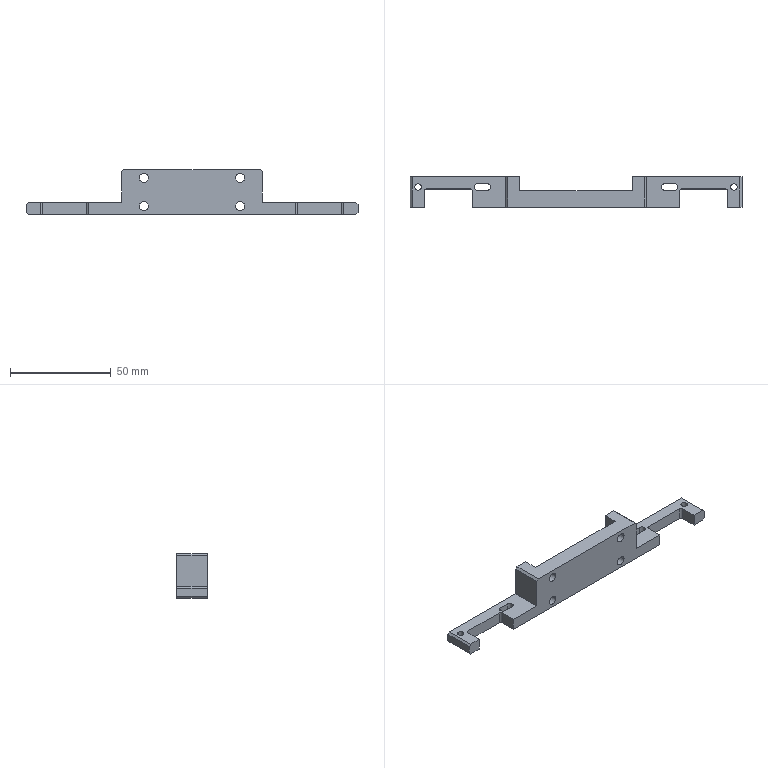Component | SolidWorks | 2018SOLIDWORKS1400000007-1 | 1 solid | 52 faces | box 165 x 15 x 22 mm | volume 19500 mm3 | plane 32 | cylinder 20 | commonest cylinder face diameters 3.2 x8 4.5 x8 2 x4 | material Bakelite
build123d program:
from build123d import *

# Parameters (mm, degrees)
SKETCH1_W                  = 165
SKETCH1_H                  = 22
BOSS_EXTRUDE1_DEPTH        = 15
SKETCH4_W                  = 56
SKETCH4_H                  = 22
CUT_EXTRUDE3_DEPTH         = 7
SKETCH5_W                  = 47.5
SKETCH5_H                  = 16
CUT_EXTRUDE4_DEPTH         = 85.571
F_4_5_4_5_DIAMETER_HOLE1_D = 4.5
CHAMFER1_SIZE              = 1
SKETCH11_R                 = 1.6
CUT_EXTRUDE5_DEPTH         = 87.691
SKETCH12_W                 = 24
SKETCH12_H                 = 9
CUT_EXTRUDE6_DEPTH         = 86.365
FILLET1_R                  = 1


with BuildPart() as part:
    # Sketch1 → Boss-Extrude1 (new body)
    with BuildSketch(Plane.XY):
        Rectangle(SKETCH1_W, SKETCH1_H)
    extrude(amount=BOSS_EXTRUDE1_DEPTH)

    # Sketch4 → Cut-Extrude3 (cut)
    with BuildSketch(Plane.XY):
        Rectangle(SKETCH4_W, SKETCH4_H)
    extrude(amount=CUT_EXTRUDE3_DEPTH, mode=Mode.SUBTRACT)

    # Sketch5 → Cut-Extrude4 (cut, through all)
    with BuildSketch(Plane.XY.offset(15)):
        with Locations((-58.75, 3)):
            Rectangle(SKETCH5_W, SKETCH5_H)
        with Locations((58.75, 3)):
            Rectangle(SKETCH5_W, SKETCH5_H)
    extrude(amount=-CUT_EXTRUDE4_DEPTH, mode=Mode.SUBTRACT)

    # 4.5 _4.5_ Diameter Hole1 (through all)
    with Locations(Plane.XY.offset(15)):
        with Locations((24, 7), (24, -7), (-24, 7), (-24, -7)):
            Hole(F_4_5_4_5_DIAMETER_HOLE1_D / 2)

    # Chamfer1
    chamfer1_edges = [part.edges().sort_by_distance(p)[0] for p in [
        (-82.5, -5, 7.5),
        (-35, 11, 7.5),
        (82.5, -5, 7.5),
        (35, 11, 7.5),
        (82.5, -11, 7.5),
        (-82.5, -11, 7.5),
    ]]
    chamfer(chamfer1_edges, length=CHAMFER1_SIZE)

    # Sketch11 → Cut-Extrude5 (cut, through all)
    with BuildSketch(Plane.XZ.offset(11)):
        with Locations(Location((-78.5, 5, 0), (0, 0, 270))):
            Circle(SKETCH11_R)
        with Locations(Location((78.5, 5, 0), (0, 0, 270))):
            Circle(SKETCH11_R)
        with BuildLine():
            Line((-49, 6.6), (-44, 6.6))
            ThreePointArc((-44, 6.6), (-42.4, 5), (-44, 3.4))
            Line((-44, 3.4), (-49, 3.4))
            ThreePointArc((-49, 3.4), (-50.6, 5), (-49, 6.6))
        make_face()
        with BuildLine():
            Line((44, 6.6), (49, 6.6))
            ThreePointArc((49, 6.6), (50.6, 5), (49, 3.4))
            Line((49, 3.4), (44, 3.4))
            ThreePointArc((44, 3.4), (42.4, 5), (44, 6.6))
        make_face()
    extrude(amount=-CUT_EXTRUDE5_DEPTH, mode=Mode.SUBTRACT)

    # Sketch12 → Cut-Extrude6 (cut, through all)
    with BuildSketch(Plane(origin=(0, -5, 0), x_dir=(1, 0, 0), z_dir=(0, 1, 0))):
        with Locations((-63.5, -10.5)):
            Rectangle(SKETCH12_W, SKETCH12_H)
        with Locations((63.5, -10.5)):
            Rectangle(SKETCH12_W, SKETCH12_H)
    extrude(amount=-CUT_EXTRUDE6_DEPTH, mode=Mode.SUBTRACT)

    # Fillet1
    fillet1_edges = [part.edges().sort_by_distance(p)[0] for p in [
        (-51.5, -8, 6),
        (-75.5, -8, 6),
        (75.5, -8, 6),
        (51.5, -8, 6),
    ]]
    fillet(fillet1_edges, radius=FILLET1_R)


solid = part.part

# Placed as in the assembly
solid = solid.moved(Location((163.212, -88.5, 222), (90, 0, 0)))